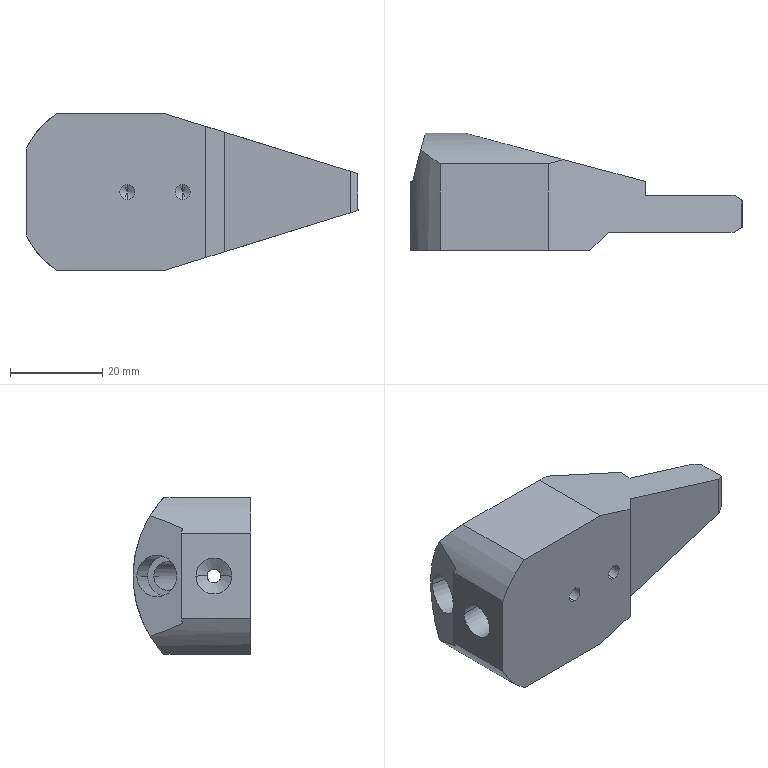Component | SolidWorks | M3Jaw-1 | 1 solid | 41 faces | volume 30902 mm3 | plane 18 | cylinder 17 | cone 6 | commonest cylinder face diameters 3.3 x4 3 x4 6.2 x2 9 x2 7.8 x2 40 x2 50 x1